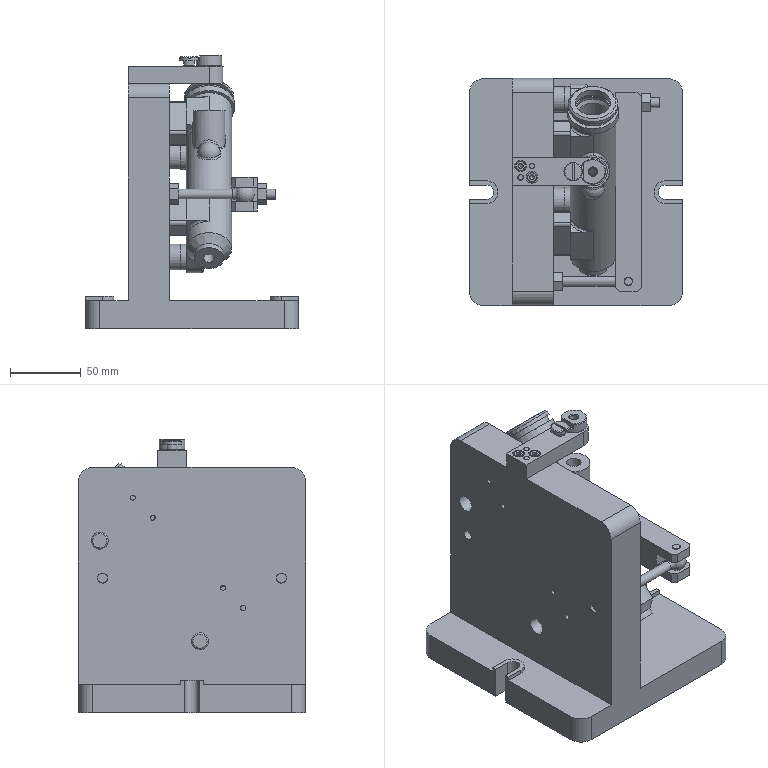Assembly | NX | mm | 21 component files | 21 solids | 437 faces | box 150 x 160 x 193 mm | volume 1362347 mm3 | plane 188 | cylinder 118 | cone 95 | spline 19 | torus 13 | sphere 4 | commonest cylinder face diameters 4 x14 6.985 x8 20 x7 13 x7 10 x6 3 x6 4.3 x6 8.3 x6
Bill of materials:
GB-T6170_F-2000,M8x1.25 | 3 |  | Hexagonal nut-like body with a central round through bore and chamfered corners on both faces.
unnamed part 1 | 1 |  | Flanged, stepped cylindrical bushing with a central through bore. The flange has a stepped lug or flat on one side, and the shank has a small neck and a chamfered end.
unnamed part 2 | 1 |  | Long rectangular bar with forked (clevis-like) slots at both ends. Cross holes are visible through the fork tines at one end, and the tine corners are chamfered.
unnamed part 3 | 1 |  | Slender cylindrical rod ending in a spherical eye with flat faces and a through hole perpendicular to the rod axis.
GB-T119.1-2000,6x24 | 1 |  | Parallel Pin, GB-T 119.1-2000,6x24
unnamed part 4 | 1 |  | Plain solid cylindrical rod with flat ends.
unnamed part 5 | 1 |  | Pin or screw with a slotted head: a chamfered round head with a straight slot, a cylindrical collar below it, a reduced neck, and a chamfered cylindrical tip.
GB-T119.1-2000,4x14 | 2 |  | Parallel Pin, GB-T 119.1-2000,4x14
unnamed part 6 | 2 |  | Rectangular plate or block with rounded corners and two round through holes, one near each end.
unnamed part 7 | 1 |  | Stepped cylindrical pin with a thin integral flange near the middle. One end is a larger chamfered cylinder; the other end is smaller and has two opposed flats and a chamfered tip.
unnamed part 8 | 1 |  | Tubular body with an open end that has a lip and groove, a perpendicular cylindrical side boss with a bore, small rounded bumps, two mounting tabs with holes, rectangular cut-outs, and a smaller bore at the closed or reduced end.
unnamed part 9 | 1 |  | Plain cylindrical sleeve or tube with a round through bore and chamfered outer edges at both ends.
unnamed part 10 | 1 |  | Thick flat link bar with one square end and one fully rounded end. It has a large through hole at the rounded end, a small hole near it, and a 2x2 pattern of four small holes at the square end.
unnamed part 11 | 1 |  | L-shaped bracket: a base plate with rounded corners and U-slots on two opposite edges, and an upright plate with several through holes of different sizes, two protruding cylindrical bosses, and a small 4-hole pattern on its top edge.
GB-T70.1-2000,M4x12 | 2 |  | Hexagon Socket Head Cap Screw, GB-T 70.1-2000,M4x12
unnamed part 12 | 1 |  | Solid stepped round pin with a thin raised collar part way along it. On each side of the collar is a short narrow neck, then a larger plain cylindrical section. Both outer ends are chamfered, and the end faces are flat.
Mates:
1. fix | fixture_body 1 component
2. touch align | spacer_block 2 face | fixture_body 1 point
3. concentric | spacer_block 2 edge | fixture_body 1 edge
4. touch align | spacer_block 1 face | fixture_body 1 face
5. concentric | spacer_block 1 edge | fixture_body 1 edge
6. concentric | loc_pin 1 edge | fixture_body 1 edge
7. concentric | loc_screw 1 edge | fixture_body 1 edge
8. touch align | workpiece 1 face | loc_screw 1 face
9. touch align | workpiece 1 face | spacer_block 1 face
10. touch align | hinge_pin 1 face | fixture_body 1 face
11. touch align | clamp_plate 1 face | hinge_pin 1 face
12. parallel | clamp_plate 1 face | fixture_body 1 face
13. touch align | clamp_plate 1 face | workpiece 1 face
14. concentric | clamp_plate 1 edge | hinge_pin 1 edge
15. touch align | screw_rod 1 face | fixture_body 1 face
16. distance | screw_rod 1 face | clamp_plate 1 face
17. touch align | GB-T6170_F-2000_M8x1_25 3 face | screw_rod 1 face
18. touch align | GB-T6170_F-2000_M8x1_25 3 face | clamp_plate 1 face
19. concentric | GB-T6170_F-2000_M8x1_25 2 edge | fixture_body 1 edge
20. concentric | GB-T6170_F-2000_M8x1_25 1 edge | fixture_body 1 edge
21. touch align | drill_template 1 face | workpiece 1 face
22. parallel | workpiece 1 face | fixture_body 1 face
23. touch align | drill_template 1 face | fixture_body 1 face
24. parallel | drill_template 1 face | fixture_body 1 face
25. concentric | bushing 1 edge | drill_template 1 edge
26. concentric | drill_bushing 1 edge | bushing 1 edge
27. touch align | drill_bushing_screw 1 face | drill_template 1 face
28. touch align | drill_bushing_screw 1 face | drill_bushing 1 face
29. concentric | GB-T70_1-2000_M4x12 1 edge | drill_template 1 edge
30. concentric | GB-T119_1-2000_4x14 2 edge | drill_template 1 edge
31. concentric | GB-T119_1-2000_4x14 1 edge | drill_template 1 edge